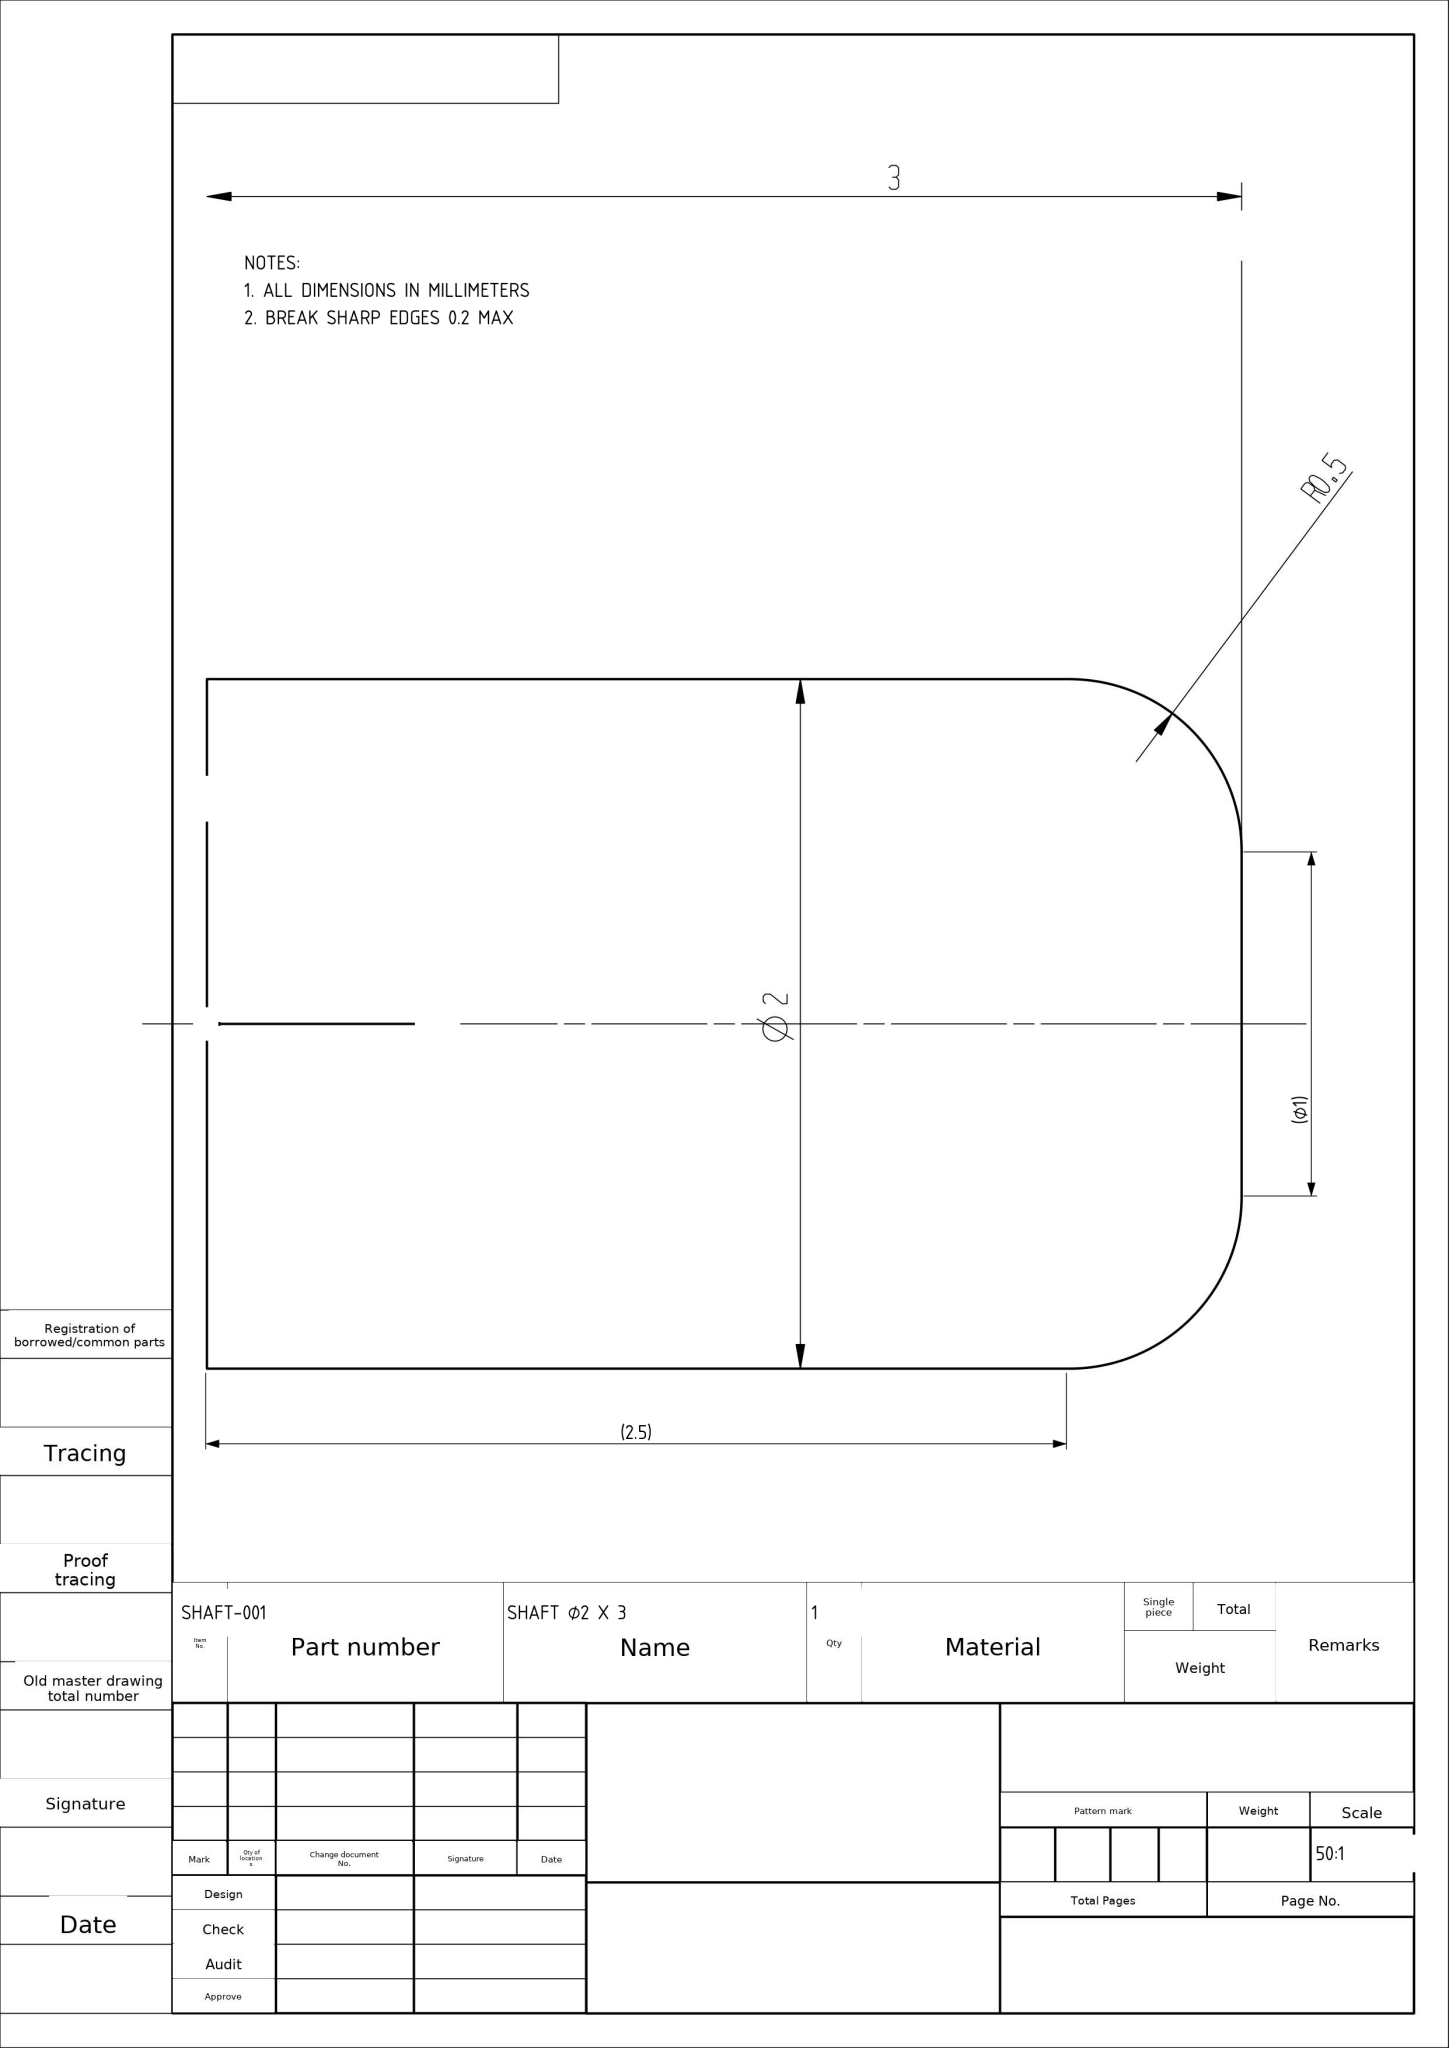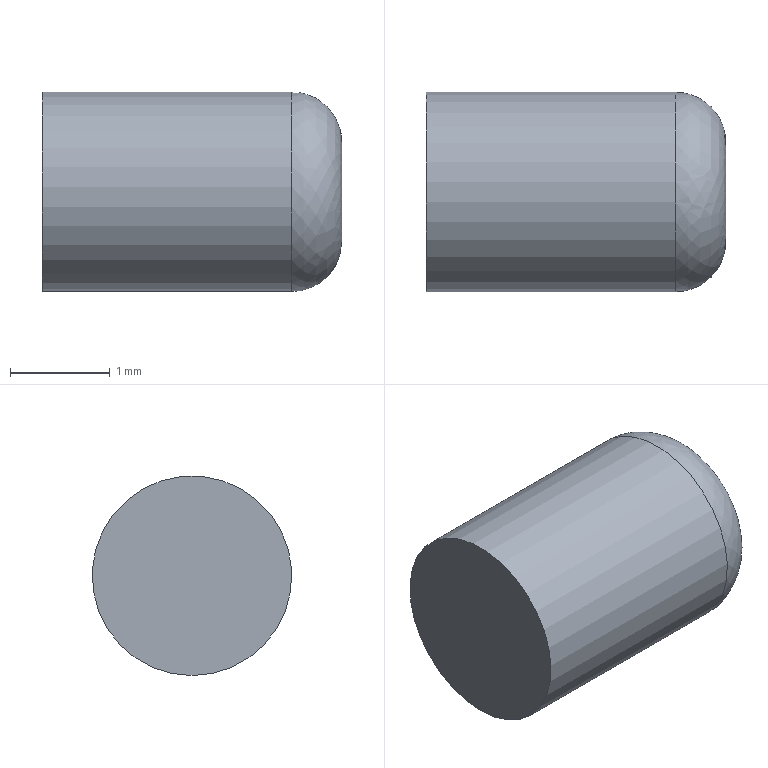Part | NX | mm | 1 solid | 4 faces | box 3 x 2 x 2 mm | volume 9 mm3 | plane 2 | cylinder 1 | spline 1 | commonest cylinder face diameters 2 x1
STEP:
#1=CARTESIAN_POINT('',(0.,0.,0.));
#2=DIRECTION('',(0.,0.,1.));
#3=DIRECTION('',(1.,0.,0.));
#4=AXIS2_PLACEMENT_3D('',#1,#2,#3);
#5=(LENGTH_UNIT()NAMED_UNIT(*)SI_UNIT(.MILLI.,.METRE.));
#6=UNCERTAINTY_MEASURE_WITH_UNIT(LENGTH_MEASURE(0.0254),#5,'','');
#7=(NAMED_UNIT(*)PLANE_ANGLE_UNIT()SI_UNIT($,.RADIAN.));
#8=PLANE_ANGLE_MEASURE_WITH_UNIT(PLANE_ANGLE_MEASURE(0.01745),#7);
#9=DIMENSIONAL_EXPONENTS(0.,0.,0.,0.,0.,0.,0.);
#10=(CONVERSION_BASED_UNIT('',#8)NAMED_UNIT(#9)PLANE_ANGLE_UNIT());
#11=(NAMED_UNIT(*)SI_UNIT($,.STERADIAN.)SOLID_ANGLE_UNIT());
#12=(GEOMETRIC_REPRESENTATION_CONTEXT(3)GLOBAL_UNCERTAINTY_ASSIGNED_CONTEXT((#6))GLOBAL_UNIT_ASSIGNED_CONTEXT((#5,#10,#11))REPRESENTATION_CONTEXT('',''));
#13=SHAPE_REPRESENTATION('',(#4),#12);
#14=CARTESIAN_POINT('',(3.,0.,-0.5));
#15=VERTEX_POINT('',#14);
#16=CARTESIAN_POINT('',(3.,0.,0.));
#17=DIRECTION('',(1.,0.,0.));
#18=DIRECTION('',(0.,0.,-1.));
#19=AXIS2_PLACEMENT_3D('',#16,#17,#18);
#20=CIRCLE('',#19,0.5);
#21=EDGE_CURVE('',#15,#15,#20,.T.);
#22=ORIENTED_EDGE('',*,*,#21,.T.);
#23=EDGE_LOOP('',(#22));
#24=FACE_OUTER_BOUND('',#23,.T.);
#25=CARTESIAN_POINT('',(3.,0.,0.));
#26=DIRECTION('',(1.,0.,0.));
#27=DIRECTION('',(0.,0.,-1.));
#28=AXIS2_PLACEMENT_3D('',#25,#26,#27);
#29=PLANE('',#28);
#30=ADVANCED_FACE('',(#24),#29,.T.);
#31=CARTESIAN_POINT('',(0.,0.,-1.));
#32=VERTEX_POINT('',#31);
#33=CARTESIAN_POINT('',(0.,0.,0.));
#34=DIRECTION('',(1.,0.,0.));
#35=DIRECTION('',(0.,0.,-1.));
#36=AXIS2_PLACEMENT_3D('',#33,#34,#35);
#37=CIRCLE('',#36,1.);
#38=EDGE_CURVE('',#32,#32,#37,.T.);
#39=ORIENTED_EDGE('',*,*,#38,.F.);
#40=EDGE_LOOP('',(#39));
#41=FACE_OUTER_BOUND('',#40,.T.);
#42=CARTESIAN_POINT('',(0.,0.,0.));
#43=DIRECTION('',(-1.,0.,0.));
#44=DIRECTION('',(0.,0.,1.));
#45=AXIS2_PLACEMENT_3D('',#42,#43,#44);
#46=PLANE('',#45);
#47=ADVANCED_FACE('',(#41),#46,.T.);
#48=CARTESIAN_POINT('',(2.5,0.,-1.));
#49=VERTEX_POINT('',#48);
#50=CARTESIAN_POINT('',(2.5,0.,0.));
#51=DIRECTION('',(-1.,0.,0.));
#52=DIRECTION('',(0.,0.,-1.));
#53=AXIS2_PLACEMENT_3D('',#50,#51,#52);
#54=CIRCLE('',#53,1.);
#55=EDGE_CURVE('',#49,#49,#54,.T.);
#56=ORIENTED_EDGE('',*,*,#55,.T.);
#57=EDGE_LOOP('',(#56));
#58=FACE_BOUND('',#57,.T.);
#59=ORIENTED_EDGE('',*,*,#38,.T.);
#60=EDGE_LOOP('',(#59));
#61=FACE_BOUND('',#60,.T.);
#62=CARTESIAN_POINT('',(0.,0.,0.));
#63=DIRECTION('',(1.,0.,0.));
#64=DIRECTION('',(0.,0.,-1.));
#65=AXIS2_PLACEMENT_3D('',#62,#63,#64);
#66=CYLINDRICAL_SURFACE('',#65,1.);
#67=ADVANCED_FACE('',(#58,#61),#66,.T.);
#68=ORIENTED_EDGE('',*,*,#21,.F.);
#69=EDGE_LOOP('',(#68));
#70=FACE_BOUND('',#69,.T.);
#71=ORIENTED_EDGE('',*,*,#55,.F.);
#72=EDGE_LOOP('',(#71));
#73=FACE_BOUND('',#72,.T.);
#74=CARTESIAN_POINT('',(3.,0.,-0.5));
#75=CARTESIAN_POINT('',(3.,1.,-0.5));
#76=CARTESIAN_POINT('',(3.,1.,0.5));
#77=CARTESIAN_POINT('',(3.,0.,0.5));
#78=CARTESIAN_POINT('',(3.,-1.,0.5));
#79=CARTESIAN_POINT('',(3.,-1.,-0.5));
#80=CARTESIAN_POINT('',(3.,0.,-0.5));
#81=CARTESIAN_POINT('',(3.,0.,-0.7929));
#82=CARTESIAN_POINT('',(3.,1.586,-0.7929));
#83=CARTESIAN_POINT('',(3.,1.586,0.7929));
#84=CARTESIAN_POINT('',(3.,0.,0.7929));
#85=CARTESIAN_POINT('',(3.,-1.586,0.7929));
#86=CARTESIAN_POINT('',(3.,-1.586,-0.7929));
#87=CARTESIAN_POINT('',(3.,0.,-0.7929));
#88=CARTESIAN_POINT('',(2.793,0.,-1.));
#89=CARTESIAN_POINT('',(2.793,2.,-1.));
#90=CARTESIAN_POINT('',(2.793,2.,1.));
#91=CARTESIAN_POINT('',(2.793,0.,1.));
#92=CARTESIAN_POINT('',(2.793,-2.,1.));
#93=CARTESIAN_POINT('',(2.793,-2.,-1.));
#94=CARTESIAN_POINT('',(2.793,0.,-1.));
#95=CARTESIAN_POINT('',(2.5,0.,-1.));
#96=CARTESIAN_POINT('',(2.5,2.,-1.));
#97=CARTESIAN_POINT('',(2.5,2.,1.));
#98=CARTESIAN_POINT('',(2.5,0.,1.));
#99=CARTESIAN_POINT('',(2.5,-2.,1.));
#100=CARTESIAN_POINT('',(2.5,-2.,-1.));
#101=CARTESIAN_POINT('',(2.5,0.,-1.));
#102=(BOUNDED_SURFACE()B_SPLINE_SURFACE(3,3,((#74,#75,#76,#77,#78,#79,#80),(#81,#82,#83,#84,#85,#86,#87),(#88,#89,#90,#91,#92,#93,#94),(#95,#96,#97,#98,#99,#100,#101)),.UNSPECIFIED.,.F.,.T.,.F.)B_SPLINE_SURFACE_WITH_KNOTS((4,4),(1,3,3,3,1),(0.,1.),(-0.5,0.,0.5,1.,1.5),.UNSPECIFIED.)GEOMETRIC_REPRESENTATION_ITEM()RATIONAL_B_SPLINE_SURFACE(((1.,0.3333,0.3333,1.,0.3333,0.3333,1.),(0.8047,0.2682,0.2682,0.8047,0.2682,0.2682,0.8047),(0.8047,0.2682,0.2682,0.8047,0.2682,0.2682,0.8047),(1.,0.3333,0.3333,1.,0.3333,0.3333,1.)))REPRESENTATION_ITEM('')SURFACE());
#103=ADVANCED_FACE('',(#70,#73),#102,.T.);
#104=CLOSED_SHELL('',(#30,#47,#67,#103));
#105=MANIFOLD_SOLID_BREP('',#104);
#106=ADVANCED_BREP_SHAPE_REPRESENTATION('',(#105),#12);
#107=SHAPE_REPRESENTATION_RELATIONSHIP('','',#13,#106);
#108=PRESENTATION_LAYER_ASSIGNMENT('','',(#105));
#109=COLOUR_RGB('',0.6941,0.6941,0.6941);
#110=FILL_AREA_STYLE_COLOUR('',#109);
#111=FILL_AREA_STYLE('',(#110));
#112=SURFACE_STYLE_FILL_AREA(#111);
#113=SURFACE_SIDE_STYLE('',(#112));
#114=SURFACE_STYLE_USAGE(.BOTH.,#113);
#115=PRESENTATION_STYLE_ASSIGNMENT((#114));
#116=STYLED_ITEM('',(#115),#105);
#117=MECHANICAL_DESIGN_GEOMETRIC_PRESENTATION_REPRESENTATION('',(#116),#12);